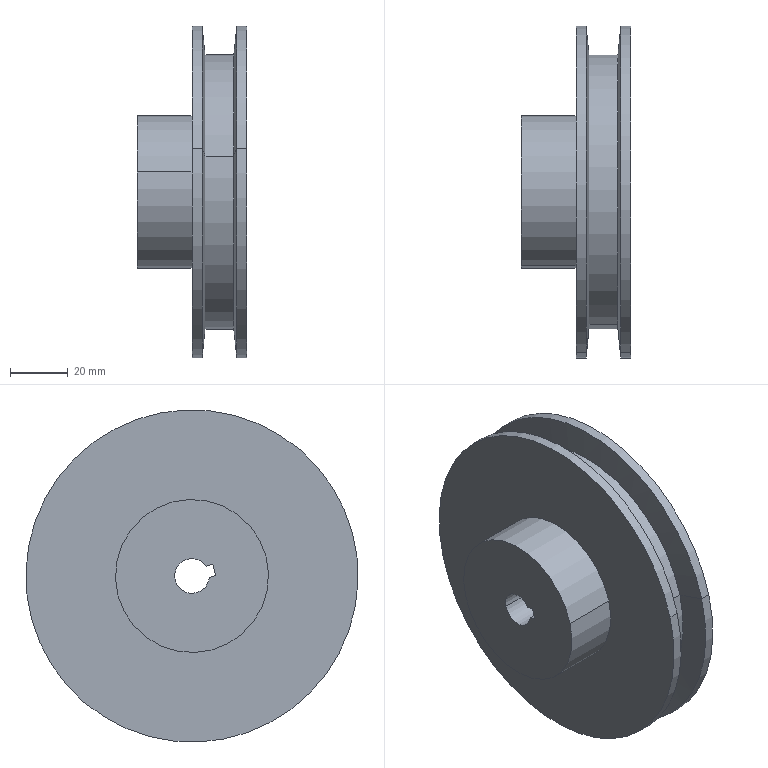Component | SolidWorks | ReducerPulley-1 | 1 solid | 23 faces | box 38 x 115 x 115 mm | volume 149209 mm3 | cylinder 12 | plane 7 | cone 4 | commonest cylinder face diameters 115 x4 12 x2 80 x2 95 x2 53 x2
build123d program:
from build123d import *

# Parameters (mm, degrees)
EXTRUDE1_DEPTH = 87.003


with BuildPart() as part:
    # Sketch1 → Revolve1 (revolve)
    with BuildSketch(Plane.XY, mode=Mode.PRIVATE) as revolve1_sk:
        Polygon((0, 26.5), (19, 26.5), (19, 57.5), (22.5, 57.5), (23.5, 47.5), (33.5, 47.5), (34.5, 57.5), (38, 57.5), (38, 40), (28, 40), (28, 6), (0, 6), align=None)
    revolve(revolve1_sk.sketch.rotate(Axis((28, 0, 0), (1, 0, 0)), 180), axis=Axis((28, 0, 0), (1, 0, 0)))

    # Sketch2 → Extrude1 (cut, through all)
    with BuildSketch(Plane(origin=(28, 0, 0), x_dir=(0, 0, -1), z_dir=(1, 0, 0))):
        Polygon((-2, 8), (2, 8), (2, 2.309), (-2, -3.772), align=None)
    extrude(amount=-EXTRUDE1_DEPTH, mode=Mode.SUBTRACT)


solid = part.part

# Placed as in the assembly
solid = solid.moved(Location((191.216, 175.983, 58.736), (164.849, 0, 0)))
STEP:
#1=COLOUR_RGB('',0.7922,0.8196,0.9333);
#2=FILL_AREA_STYLE_COLOUR('',#1);
#3=FILL_AREA_STYLE('',(#2));
#4=SURFACE_STYLE_FILL_AREA(#3);
#5=SURFACE_SIDE_STYLE('',(#4));
#6=SURFACE_STYLE_USAGE(.BOTH.,#5);
#7=PRESENTATION_STYLE_ASSIGNMENT((#6));
#8=CARTESIAN_POINT('',(8.631,7.156,2.251));
#9=VERTEX_POINT('',#8);
#10=CARTESIAN_POINT('',(8.631,6.693,2.295));
#11=VERTEX_POINT('',#10);
#12=CARTESIAN_POINT('',(8.631,6.928,2.312));
#13=DIRECTION('',(-1.,0.,-0.));
#14=DIRECTION('',(0.,0.9652,-0.2614));
#15=AXIS2_PLACEMENT_3D('',#12,#13,#14);
#16=CIRCLE('',#15,0.2362);
#17=EDGE_CURVE('',#9,#11,#16,.T.);
#18=ORIENTED_EDGE('',*,*,#17,.F.);
#19=CARTESIAN_POINT('',(7.528,7.156,2.251));
#20=VERTEX_POINT('',#19);
#21=CARTESIAN_POINT('',(8.631,7.156,2.251));
#22=DIRECTION('',(-1.,0.,-0.));
#23=VECTOR('',#22,39.37);
#24=LINE('',#21,#23);
#25=EDGE_CURVE('',#9,#20,#24,.T.);
#26=ORIENTED_EDGE('',*,*,#25,.T.);
#27=CARTESIAN_POINT('',(7.528,6.693,2.295));
#28=VERTEX_POINT('',#27);
#29=CARTESIAN_POINT('',(7.528,6.928,2.312));
#30=DIRECTION('',(-1.,0.,-0.));
#31=DIRECTION('',(0.,0.9652,-0.2614));
#32=AXIS2_PLACEMENT_3D('',#29,#30,#31);
#33=CIRCLE('',#32,0.2362);
#34=EDGE_CURVE('',#20,#28,#33,.T.);
#35=ORIENTED_EDGE('',*,*,#34,.T.);
#36=CARTESIAN_POINT('',(8.631,6.693,2.295));
#37=DIRECTION('',(1.,-0.,0.));
#38=VECTOR('',#37,39.37);
#39=LINE('',#36,#38);
#40=EDGE_CURVE('',#28,#11,#39,.T.);
#41=ORIENTED_EDGE('',*,*,#40,.T.);
#42=EDGE_LOOP('',(#18,#26,#35,#41));
#43=FACE_OUTER_BOUND('',#42,.T.);
#44=CARTESIAN_POINT('',(8.631,6.928,2.312));
#45=DIRECTION('',(-1.,0.,-0.));
#46=DIRECTION('',(0.,0.9652,-0.2614));
#47=AXIS2_PLACEMENT_3D('',#44,#45,#46);
#48=CYLINDRICAL_SURFACE('',#47,0.2362);
#49=ADVANCED_FACE('',(#43),#48,.F.);
#50=CARTESIAN_POINT('',(9.024,5.408,2.724));
#51=VERTEX_POINT('',#50);
#52=CARTESIAN_POINT('',(9.024,8.449,1.901));
#53=VERTEX_POINT('',#52);
#54=CARTESIAN_POINT('',(9.024,6.928,2.312));
#55=DIRECTION('',(-1.,0.,-0.));
#56=DIRECTION('',(0.,0.9652,-0.2614));
#57=AXIS2_PLACEMENT_3D('',#54,#55,#56);
#58=CIRCLE('',#57,1.575);
#59=EDGE_CURVE('',#51,#53,#58,.T.);
#60=ORIENTED_EDGE('',*,*,#59,.F.);
#61=CARTESIAN_POINT('',(8.631,5.408,2.724));
#62=VERTEX_POINT('',#61);
#63=CARTESIAN_POINT('',(8.631,5.408,2.724));
#64=DIRECTION('',(-1.,0.,-0.));
#65=VECTOR('',#64,39.37);
#66=LINE('',#63,#65);
#67=EDGE_CURVE('',#51,#62,#66,.T.);
#68=ORIENTED_EDGE('',*,*,#67,.T.);
#69=CARTESIAN_POINT('',(8.631,8.449,1.901));
#70=VERTEX_POINT('',#69);
#71=CARTESIAN_POINT('',(8.631,6.928,2.312));
#72=DIRECTION('',(-1.,0.,-0.));
#73=DIRECTION('',(0.,0.9652,-0.2614));
#74=AXIS2_PLACEMENT_3D('',#71,#72,#73);
#75=CIRCLE('',#74,1.575);
#76=EDGE_CURVE('',#62,#70,#75,.T.);
#77=ORIENTED_EDGE('',*,*,#76,.T.);
#78=CARTESIAN_POINT('',(8.631,8.449,1.901));
#79=DIRECTION('',(-1.,0.,-0.));
#80=VECTOR('',#79,39.37);
#81=LINE('',#78,#80);
#82=EDGE_CURVE('',#53,#70,#81,.T.);
#83=ORIENTED_EDGE('',*,*,#82,.F.);
#84=EDGE_LOOP('',(#60,#68,#77,#83));
#85=FACE_OUTER_BOUND('',#84,.T.);
#86=CARTESIAN_POINT('',(8.631,6.928,2.312));
#87=DIRECTION('',(-1.,0.,-0.));
#88=DIRECTION('',(0.,0.9652,-0.2614));
#89=AXIS2_PLACEMENT_3D('',#86,#87,#88);
#90=CYLINDRICAL_SURFACE('',#89,1.575);
#91=ADVANCED_FACE('',(#85),#90,.F.);
#92=CARTESIAN_POINT('',(9.024,9.114,1.721));
#93=VERTEX_POINT('',#92);
#94=CARTESIAN_POINT('',(9.024,4.743,2.904));
#95=VERTEX_POINT('',#94);
#96=CARTESIAN_POINT('',(9.024,6.928,2.312));
#97=DIRECTION('',(-1.,0.,-0.));
#98=DIRECTION('',(0.,0.9652,-0.2614));
#99=AXIS2_PLACEMENT_3D('',#96,#97,#98);
#100=CIRCLE('',#99,2.264);
#101=EDGE_CURVE('',#93,#95,#100,.T.);
#102=ORIENTED_EDGE('',*,*,#101,.T.);
#103=CARTESIAN_POINT('',(8.886,4.743,2.904));
#104=VERTEX_POINT('',#103);
#105=CARTESIAN_POINT('',(8.631,4.743,2.904));
#106=DIRECTION('',(-1.,0.,-0.));
#107=VECTOR('',#106,39.37);
#108=LINE('',#105,#107);
#109=EDGE_CURVE('',#95,#104,#108,.T.);
#110=ORIENTED_EDGE('',*,*,#109,.T.);
#111=CARTESIAN_POINT('',(8.886,9.114,1.721));
#112=VERTEX_POINT('',#111);
#113=CARTESIAN_POINT('',(8.886,6.928,2.312));
#114=DIRECTION('',(-1.,0.,-0.));
#115=DIRECTION('',(0.,0.9652,-0.2614));
#116=AXIS2_PLACEMENT_3D('',#113,#114,#115);
#117=CIRCLE('',#116,2.264);
#118=EDGE_CURVE('',#112,#104,#117,.T.);
#119=ORIENTED_EDGE('',*,*,#118,.F.);
#120=CARTESIAN_POINT('',(8.631,9.114,1.721));
#121=DIRECTION('',(-1.,0.,-0.));
#122=VECTOR('',#121,39.37);
#123=LINE('',#120,#122);
#124=EDGE_CURVE('',#93,#112,#123,.T.);
#125=ORIENTED_EDGE('',*,*,#124,.F.);
#126=EDGE_LOOP('',(#102,#110,#119,#125));
#127=FACE_OUTER_BOUND('',#126,.T.);
#128=CARTESIAN_POINT('',(8.631,6.928,2.312));
#129=DIRECTION('',(-1.,0.,-0.));
#130=DIRECTION('',(0.,0.9652,-0.2614));
#131=AXIS2_PLACEMENT_3D('',#128,#129,#130);
#132=CYLINDRICAL_SURFACE('',#131,2.264);
#133=ADVANCED_FACE('',(#127),#132,.T.);
#134=CARTESIAN_POINT('',(8.847,8.734,1.824));
#135=VERTEX_POINT('',#134);
#136=CARTESIAN_POINT('',(8.847,5.123,2.801));
#137=VERTEX_POINT('',#136);
#138=CARTESIAN_POINT('',(8.847,6.928,2.312));
#139=DIRECTION('',(-1.,0.,-0.));
#140=DIRECTION('',(0.,0.9652,-0.2614));
#141=AXIS2_PLACEMENT_3D('',#138,#139,#140);
#142=CIRCLE('',#141,1.87);
#143=EDGE_CURVE('',#135,#137,#142,.T.);
#144=ORIENTED_EDGE('',*,*,#143,.F.);
#145=CARTESIAN_POINT('',(8.886,9.114,1.721));
#146=DIRECTION('',(0.0995,0.9604,-0.2601));
#147=VECTOR('',#146,39.37);
#148=LINE('',#145,#147);
#149=EDGE_CURVE('',#135,#112,#148,.T.);
#150=ORIENTED_EDGE('',*,*,#149,.T.);
#151=ORIENTED_EDGE('',*,*,#118,.T.);
#152=CARTESIAN_POINT('',(8.886,4.743,2.904));
#153=DIRECTION('',(0.0995,-0.9604,0.2601));
#154=VECTOR('',#153,39.37);
#155=LINE('',#152,#154);
#156=EDGE_CURVE('',#137,#104,#155,.T.);
#157=ORIENTED_EDGE('',*,*,#156,.F.);
#158=EDGE_LOOP('',(#144,#150,#151,#157));
#159=FACE_OUTER_BOUND('',#158,.T.);
#160=CARTESIAN_POINT('',(8.886,6.928,2.312));
#161=DIRECTION('',(1.,-0.,0.));
#162=DIRECTION('',(0.,-0.9652,0.2614));
#163=AXIS2_PLACEMENT_3D('',#160,#161,#162);
#164=CONICAL_SURFACE('',#163,2.264,1.471);
#165=ADVANCED_FACE('',(#159),#164,.T.);
#166=ORIENTED_EDGE('',*,*,#143,.T.);
#167=CARTESIAN_POINT('',(8.453,5.123,2.801));
#168=VERTEX_POINT('',#167);
#169=CARTESIAN_POINT('',(8.631,5.123,2.801));
#170=DIRECTION('',(-1.,0.,-0.));
#171=VECTOR('',#170,39.37);
#172=LINE('',#169,#171);
#173=EDGE_CURVE('',#137,#168,#172,.T.);
#174=ORIENTED_EDGE('',*,*,#173,.T.);
#175=CARTESIAN_POINT('',(8.453,8.734,1.824));
#176=VERTEX_POINT('',#175);
#177=CARTESIAN_POINT('',(8.453,6.928,2.312));
#178=DIRECTION('',(-1.,0.,-0.));
#179=DIRECTION('',(0.,0.9652,-0.2614));
#180=AXIS2_PLACEMENT_3D('',#177,#178,#179);
#181=CIRCLE('',#180,1.87);
#182=EDGE_CURVE('',#176,#168,#181,.T.);
#183=ORIENTED_EDGE('',*,*,#182,.F.);
#184=CARTESIAN_POINT('',(8.631,8.734,1.824));
#185=DIRECTION('',(-1.,0.,-0.));
#186=VECTOR('',#185,39.37);
#187=LINE('',#184,#186);
#188=EDGE_CURVE('',#135,#176,#187,.T.);
#189=ORIENTED_EDGE('',*,*,#188,.F.);
#190=EDGE_LOOP('',(#166,#174,#183,#189));
#191=FACE_OUTER_BOUND('',#190,.T.);
#192=CARTESIAN_POINT('',(8.631,6.928,2.312));
#193=DIRECTION('',(-1.,0.,-0.));
#194=DIRECTION('',(0.,0.9652,-0.2614));
#195=AXIS2_PLACEMENT_3D('',#192,#193,#194);
#196=CYLINDRICAL_SURFACE('',#195,1.87);
#197=ADVANCED_FACE('',(#191),#196,.T.);
#198=ORIENTED_EDGE('',*,*,#182,.T.);
#199=CARTESIAN_POINT('',(8.414,4.743,2.904));
#200=VERTEX_POINT('',#199);
#201=CARTESIAN_POINT('',(8.453,5.123,2.801));
#202=DIRECTION('',(-0.0995,-0.9604,0.2601));
#203=VECTOR('',#202,39.37);
#204=LINE('',#201,#203);
#205=EDGE_CURVE('',#168,#200,#204,.T.);
#206=ORIENTED_EDGE('',*,*,#205,.T.);
#207=CARTESIAN_POINT('',(8.414,9.114,1.721));
#208=VERTEX_POINT('',#207);
#209=CARTESIAN_POINT('',(8.414,6.928,2.312));
#210=DIRECTION('',(-1.,0.,-0.));
#211=DIRECTION('',(0.,0.9652,-0.2614));
#212=AXIS2_PLACEMENT_3D('',#209,#210,#211);
#213=CIRCLE('',#212,2.264);
#214=EDGE_CURVE('',#208,#200,#213,.T.);
#215=ORIENTED_EDGE('',*,*,#214,.F.);
#216=CARTESIAN_POINT('',(8.453,8.734,1.824));
#217=DIRECTION('',(-0.0995,0.9604,-0.2601));
#218=VECTOR('',#217,39.37);
#219=LINE('',#216,#218);
#220=EDGE_CURVE('',#176,#208,#219,.T.);
#221=ORIENTED_EDGE('',*,*,#220,.F.);
#222=EDGE_LOOP('',(#198,#206,#215,#221));
#223=FACE_OUTER_BOUND('',#222,.T.);
#224=CARTESIAN_POINT('',(8.453,6.928,2.312));
#225=DIRECTION('',(-1.,0.,-0.));
#226=DIRECTION('',(0.,0.9652,-0.2614));
#227=AXIS2_PLACEMENT_3D('',#224,#225,#226);
#228=CONICAL_SURFACE('',#227,1.87,1.471);
#229=ADVANCED_FACE('',(#223),#228,.T.);
#230=ORIENTED_EDGE('',*,*,#214,.T.);
#231=CARTESIAN_POINT('',(8.276,4.743,2.904));
#232=VERTEX_POINT('',#231);
#233=CARTESIAN_POINT('',(8.631,4.743,2.904));
#234=DIRECTION('',(-1.,0.,-0.));
#235=VECTOR('',#234,39.37);
#236=LINE('',#233,#235);
#237=EDGE_CURVE('',#200,#232,#236,.T.);
#238=ORIENTED_EDGE('',*,*,#237,.T.);
#239=CARTESIAN_POINT('',(8.276,9.114,1.721));
#240=VERTEX_POINT('',#239);
#241=CARTESIAN_POINT('',(8.276,6.928,2.312));
#242=DIRECTION('',(-1.,0.,-0.));
#243=DIRECTION('',(0.,0.9652,-0.2614));
#244=AXIS2_PLACEMENT_3D('',#241,#242,#243);
#245=CIRCLE('',#244,2.264);
#246=EDGE_CURVE('',#240,#232,#245,.T.);
#247=ORIENTED_EDGE('',*,*,#246,.F.);
#248=CARTESIAN_POINT('',(8.631,9.114,1.721));
#249=DIRECTION('',(-1.,0.,-0.));
#250=VECTOR('',#249,39.37);
#251=LINE('',#248,#250);
#252=EDGE_CURVE('',#208,#240,#251,.T.);
#253=ORIENTED_EDGE('',*,*,#252,.F.);
#254=EDGE_LOOP('',(#230,#238,#247,#253));
#255=FACE_OUTER_BOUND('',#254,.T.);
#256=CARTESIAN_POINT('',(8.631,6.928,2.312));
#257=DIRECTION('',(-1.,0.,-0.));
#258=DIRECTION('',(0.,0.9652,-0.2614));
#259=AXIS2_PLACEMENT_3D('',#256,#257,#258);
#260=CYLINDRICAL_SURFACE('',#259,2.264);
#261=ADVANCED_FACE('',(#255),#260,.T.);
#262=CARTESIAN_POINT('',(8.276,7.936,2.04));
#263=VERTEX_POINT('',#262);
#264=CARTESIAN_POINT('',(8.276,5.921,2.585));
#265=VERTEX_POINT('',#264);
#266=CARTESIAN_POINT('',(8.276,6.928,2.312));
#267=DIRECTION('',(-1.,0.,-0.));
#268=DIRECTION('',(0.,0.9652,-0.2614));
#269=AXIS2_PLACEMENT_3D('',#266,#267,#268);
#270=CIRCLE('',#269,1.043);
#271=EDGE_CURVE('',#263,#265,#270,.T.);
#272=ORIENTED_EDGE('',*,*,#271,.T.);
#273=CARTESIAN_POINT('',(7.528,5.921,2.585));
#274=VERTEX_POINT('',#273);
#275=CARTESIAN_POINT('',(8.631,5.921,2.585));
#276=DIRECTION('',(-1.,0.,-0.));
#277=VECTOR('',#276,39.37);
#278=LINE('',#275,#277);
#279=EDGE_CURVE('',#265,#274,#278,.T.);
#280=ORIENTED_EDGE('',*,*,#279,.T.);
#281=CARTESIAN_POINT('',(7.528,7.936,2.04));
#282=VERTEX_POINT('',#281);
#283=CARTESIAN_POINT('',(7.528,6.928,2.312));
#284=DIRECTION('',(-1.,0.,-0.));
#285=DIRECTION('',(0.,0.9652,-0.2614));
#286=AXIS2_PLACEMENT_3D('',#283,#284,#285);
#287=CIRCLE('',#286,1.043);
#288=EDGE_CURVE('',#282,#274,#287,.T.);
#289=ORIENTED_EDGE('',*,*,#288,.F.);
#290=CARTESIAN_POINT('',(8.631,7.936,2.04));
#291=DIRECTION('',(-1.,0.,-0.));
#292=VECTOR('',#291,39.37);
#293=LINE('',#290,#292);
#294=EDGE_CURVE('',#263,#282,#293,.T.);
#295=ORIENTED_EDGE('',*,*,#294,.F.);
#296=EDGE_LOOP('',(#272,#280,#289,#295));
#297=FACE_OUTER_BOUND('',#296,.T.);
#298=CARTESIAN_POINT('',(8.631,6.928,2.312));
#299=DIRECTION('',(-1.,0.,-0.));
#300=DIRECTION('',(0.,0.9652,-0.2614));
#301=AXIS2_PLACEMENT_3D('',#298,#299,#300);
#302=CYLINDRICAL_SURFACE('',#301,1.043);
#303=ADVANCED_FACE('',(#297),#302,.T.);
#304=CARTESIAN_POINT('',(7.528,6.645,2.471));
#305=VERTEX_POINT('',#304);
#306=CARTESIAN_POINT('',(7.528,6.604,2.319));
#307=VERTEX_POINT('',#306);
#308=CARTESIAN_POINT('',(7.528,6.604,2.319));
#309=DIRECTION('',(-0.,-0.2614,-0.9652));
#310=VECTOR('',#309,39.37);
#311=LINE('',#308,#310);
#312=EDGE_CURVE('',#305,#307,#311,.T.);
#313=ORIENTED_EDGE('',*,*,#312,.T.);
#314=CARTESIAN_POINT('',(7.528,6.604,2.319));
#315=DIRECTION('',(0.,0.9652,-0.2614));
#316=VECTOR('',#315,39.37);
#317=LINE('',#314,#316);
#318=EDGE_CURVE('',#307,#28,#317,.T.);
#319=ORIENTED_EDGE('',*,*,#318,.T.);
#320=ORIENTED_EDGE('',*,*,#34,.F.);
#321=CARTESIAN_POINT('',(7.528,6.734,2.447));
#322=VERTEX_POINT('',#321);
#323=CARTESIAN_POINT('',(7.528,6.928,2.312));
#324=DIRECTION('',(-1.,0.,-0.));
#325=DIRECTION('',(0.,0.9652,-0.2614));
#326=AXIS2_PLACEMENT_3D('',#323,#324,#325);
#327=CIRCLE('',#326,0.2362);
#328=EDGE_CURVE('',#322,#20,#327,.T.);
#329=ORIENTED_EDGE('',*,*,#328,.F.);
#330=CARTESIAN_POINT('',(7.528,6.645,2.471));
#331=DIRECTION('',(-0.,-0.9652,0.2614));
#332=VECTOR('',#331,39.37);
#333=LINE('',#330,#332);
#334=EDGE_CURVE('',#322,#305,#333,.T.);
#335=ORIENTED_EDGE('',*,*,#334,.T.);
#336=EDGE_LOOP('',(#313,#319,#320,#329,#335));
#337=FACE_BOUND('',#336,.T.);
#338=ORIENTED_EDGE('',*,*,#288,.T.);
#339=CARTESIAN_POINT('',(7.528,6.928,2.312));
#340=DIRECTION('',(-1.,0.,-0.));
#341=DIRECTION('',(0.,0.9652,-0.2614));
#342=AXIS2_PLACEMENT_3D('',#339,#340,#341);
#343=CIRCLE('',#342,1.043);
#344=EDGE_CURVE('',#274,#282,#343,.T.);
#345=ORIENTED_EDGE('',*,*,#344,.T.);
#346=EDGE_LOOP('',(#338,#345));
#347=FACE_OUTER_BOUND('',#346,.T.);
#348=CARTESIAN_POINT('',(7.528,6.7,2.374));
#349=DIRECTION('',(1.,-0.,0.));
#350=DIRECTION('',(-0.,-0.9652,0.2614));
#351=AXIS2_PLACEMENT_3D('',#348,#349,#350);
#352=PLANE('',#351);
#353=ADVANCED_FACE('',(#337,#347),#352,.F.);
#354=ORIENTED_EDGE('',*,*,#279,.F.);
#355=CARTESIAN_POINT('',(8.276,6.928,2.312));
#356=DIRECTION('',(-1.,0.,-0.));
#357=DIRECTION('',(0.,0.9652,-0.2614));
#358=AXIS2_PLACEMENT_3D('',#355,#356,#357);
#359=CIRCLE('',#358,1.043);
#360=EDGE_CURVE('',#265,#263,#359,.T.);
#361=ORIENTED_EDGE('',*,*,#360,.T.);
#362=ORIENTED_EDGE('',*,*,#294,.T.);
#363=ORIENTED_EDGE('',*,*,#344,.F.);
#364=EDGE_LOOP('',(#354,#361,#362,#363));
#365=FACE_OUTER_BOUND('',#364,.T.);
#366=CARTESIAN_POINT('',(8.631,6.928,2.312));
#367=DIRECTION('',(-1.,0.,-0.));
#368=DIRECTION('',(0.,0.9652,-0.2614));
#369=AXIS2_PLACEMENT_3D('',#366,#367,#368);
#370=CYLINDRICAL_SURFACE('',#369,1.043);
#371=ADVANCED_FACE('',(#365),#370,.T.);
#372=ORIENTED_EDGE('',*,*,#271,.F.);
#373=ORIENTED_EDGE('',*,*,#360,.F.);
#374=EDGE_LOOP('',(#372,#373));
#375=FACE_BOUND('',#374,.T.);
#376=ORIENTED_EDGE('',*,*,#246,.T.);
#377=CARTESIAN_POINT('',(8.276,6.928,2.312));
#378=DIRECTION('',(-1.,0.,-0.));
#379=DIRECTION('',(0.,0.9652,-0.2614));
#380=AXIS2_PLACEMENT_3D('',#377,#378,#379);
#381=CIRCLE('',#380,2.264);
#382=EDGE_CURVE('',#232,#240,#381,.T.);
#383=ORIENTED_EDGE('',*,*,#382,.T.);
#384=EDGE_LOOP('',(#376,#383));
#385=FACE_OUTER_BOUND('',#384,.T.);
#386=CARTESIAN_POINT('',(8.276,5.921,2.585));
#387=DIRECTION('',(1.,-0.,0.));
#388=DIRECTION('',(-0.,-0.9652,0.2614));
#389=AXIS2_PLACEMENT_3D('',#386,#387,#388);
#390=PLANE('',#389);
#391=ADVANCED_FACE('',(#375,#385),#390,.F.);
#392=ORIENTED_EDGE('',*,*,#237,.F.);
#393=CARTESIAN_POINT('',(8.414,6.928,2.312));
#394=DIRECTION('',(-1.,0.,-0.));
#395=DIRECTION('',(0.,0.9652,-0.2614));
#396=AXIS2_PLACEMENT_3D('',#393,#394,#395);
#397=CIRCLE('',#396,2.264);
#398=EDGE_CURVE('',#200,#208,#397,.T.);
#399=ORIENTED_EDGE('',*,*,#398,.T.);
#400=ORIENTED_EDGE('',*,*,#252,.T.);
#401=ORIENTED_EDGE('',*,*,#382,.F.);
#402=EDGE_LOOP('',(#392,#399,#400,#401));
#403=FACE_OUTER_BOUND('',#402,.T.);
#404=CARTESIAN_POINT('',(8.631,6.928,2.312));
#405=DIRECTION('',(-1.,0.,-0.));
#406=DIRECTION('',(0.,0.9652,-0.2614));
#407=AXIS2_PLACEMENT_3D('',#404,#405,#406);
#408=CYLINDRICAL_SURFACE('',#407,2.264);
#409=ADVANCED_FACE('',(#403),#408,.T.);
#410=ORIENTED_EDGE('',*,*,#205,.F.);
#411=CARTESIAN_POINT('',(8.453,6.928,2.312));
#412=DIRECTION('',(-1.,0.,-0.));
#413=DIRECTION('',(0.,0.9652,-0.2614));
#414=AXIS2_PLACEMENT_3D('',#411,#412,#413);
#415=CIRCLE('',#414,1.87);
#416=EDGE_CURVE('',#168,#176,#415,.T.);
#417=ORIENTED_EDGE('',*,*,#416,.T.);
#418=ORIENTED_EDGE('',*,*,#220,.T.);
#419=ORIENTED_EDGE('',*,*,#398,.F.);
#420=EDGE_LOOP('',(#410,#417,#418,#419));
#421=FACE_OUTER_BOUND('',#420,.T.);
#422=CARTESIAN_POINT('',(8.453,6.928,2.312));
#423=DIRECTION('',(-1.,0.,-0.));
#424=DIRECTION('',(0.,0.9652,-0.2614));
#425=AXIS2_PLACEMENT_3D('',#422,#423,#424);
#426=CONICAL_SURFACE('',#425,1.87,1.471);
#427=ADVANCED_FACE('',(#421),#426,.T.);
#428=ORIENTED_EDGE('',*,*,#173,.F.);
#429=CARTESIAN_POINT('',(8.847,6.928,2.312));
#430=DIRECTION('',(-1.,0.,-0.));
#431=DIRECTION('',(0.,0.9652,-0.2614));
#432=AXIS2_PLACEMENT_3D('',#429,#430,#431);
#433=CIRCLE('',#432,1.87);
#434=EDGE_CURVE('',#137,#135,#433,.T.);
#435=ORIENTED_EDGE('',*,*,#434,.T.);
#436=ORIENTED_EDGE('',*,*,#188,.T.);
#437=ORIENTED_EDGE('',*,*,#416,.F.);
#438=EDGE_LOOP('',(#428,#435,#436,#437));
#439=FACE_OUTER_BOUND('',#438,.T.);
#440=CARTESIAN_POINT('',(8.631,6.928,2.312));
#441=DIRECTION('',(-1.,0.,-0.));
#442=DIRECTION('',(0.,0.9652,-0.2614));
#443=AXIS2_PLACEMENT_3D('',#440,#441,#442);
#444=CYLINDRICAL_SURFACE('',#443,1.87);
#445=ADVANCED_FACE('',(#439),#444,.T.);
#446=ORIENTED_EDGE('',*,*,#149,.F.);
#447=ORIENTED_EDGE('',*,*,#434,.F.);
#448=ORIENTED_EDGE('',*,*,#156,.T.);
#449=CARTESIAN_POINT('',(8.886,6.928,2.312));
#450=DIRECTION('',(-1.,0.,-0.));
#451=DIRECTION('',(0.,0.9652,-0.2614));
#452=AXIS2_PLACEMENT_3D('',#449,#450,#451);
#453=CIRCLE('',#452,2.264);
#454=EDGE_CURVE('',#104,#112,#453,.T.);
#455=ORIENTED_EDGE('',*,*,#454,.T.);
#456=EDGE_LOOP('',(#446,#447,#448,#455));
#457=FACE_OUTER_BOUND('',#456,.T.);
#458=CARTESIAN_POINT('',(8.886,6.928,2.312));
#459=DIRECTION('',(1.,-0.,0.));
#460=DIRECTION('',(0.,-0.9652,0.2614));
#461=AXIS2_PLACEMENT_3D('',#458,#459,#460);
#462=CONICAL_SURFACE('',#461,2.264,1.471);
#463=ADVANCED_FACE('',(#457),#462,.T.);
#464=ORIENTED_EDGE('',*,*,#109,.F.);
#465=CARTESIAN_POINT('',(9.024,6.928,2.312));
#466=DIRECTION('',(-1.,0.,-0.));
#467=DIRECTION('',(0.,0.9652,-0.2614));
#468=AXIS2_PLACEMENT_3D('',#465,#466,#467);
#469=CIRCLE('',#468,2.264);
#470=EDGE_CURVE('',#95,#93,#469,.T.);
#471=ORIENTED_EDGE('',*,*,#470,.T.);
#472=ORIENTED_EDGE('',*,*,#124,.T.);
#473=ORIENTED_EDGE('',*,*,#454,.F.);
#474=EDGE_LOOP('',(#464,#471,#472,#473));
#475=FACE_OUTER_BOUND('',#474,.T.);
#476=CARTESIAN_POINT('',(8.631,6.928,2.312));
#477=DIRECTION('',(-1.,0.,-0.));
#478=DIRECTION('',(0.,0.9652,-0.2614));
#479=AXIS2_PLACEMENT_3D('',#476,#477,#478);
#480=CYLINDRICAL_SURFACE('',#479,2.264);
#481=ADVANCED_FACE('',(#475),#480,.T.);
#482=ORIENTED_EDGE('',*,*,#101,.F.);
#483=ORIENTED_EDGE('',*,*,#470,.F.);
#484=EDGE_LOOP('',(#482,#483));
#485=FACE_OUTER_BOUND('',#484,.T.);
#486=CARTESIAN_POINT('',(9.024,6.928,2.312));
#487=DIRECTION('',(-1.,0.,-0.));
#488=DIRECTION('',(0.,0.9652,-0.2614));
#489=AXIS2_PLACEMENT_3D('',#486,#487,#488);
#490=CIRCLE('',#489,1.575);
#491=EDGE_CURVE('',#53,#51,#490,.T.);
#492=ORIENTED_EDGE('',*,*,#491,.T.);
#493=ORIENTED_EDGE('',*,*,#59,.T.);
#494=EDGE_LOOP('',(#492,#493));
#495=FACE_BOUND('',#494,.T.);
#496=CARTESIAN_POINT('',(9.024,4.743,2.904));
#497=DIRECTION('',(-1.,0.,-0.));
#498=DIRECTION('',(0.,0.9652,-0.2614));
#499=AXIS2_PLACEMENT_3D('',#496,#497,#498);
#500=PLANE('',#499);
#501=ADVANCED_FACE('',(#485,#495),#500,.F.);
#502=ORIENTED_EDGE('',*,*,#67,.F.);
#503=ORIENTED_EDGE('',*,*,#491,.F.);
#504=ORIENTED_EDGE('',*,*,#82,.T.);
#505=CARTESIAN_POINT('',(8.631,6.928,2.312));
#506=DIRECTION('',(-1.,0.,-0.));
#507=DIRECTION('',(0.,0.9652,-0.2614));
#508=AXIS2_PLACEMENT_3D('',#505,#506,#507);
#509=CIRCLE('',#508,1.575);
#510=EDGE_CURVE('',#70,#62,#509,.T.);
#511=ORIENTED_EDGE('',*,*,#510,.T.);
#512=EDGE_LOOP('',(#502,#503,#504,#511));
#513=FACE_OUTER_BOUND('',#512,.T.);
#514=CARTESIAN_POINT('',(8.631,6.928,2.312));
#515=DIRECTION('',(-1.,0.,-0.));
#516=DIRECTION('',(0.,0.9652,-0.2614));
#517=AXIS2_PLACEMENT_3D('',#514,#515,#516);
#518=CYLINDRICAL_SURFACE('',#517,1.575);
#519=ADVANCED_FACE('',(#513),#518,.F.);
#520=ORIENTED_EDGE('',*,*,#510,.F.);
#521=ORIENTED_EDGE('',*,*,#76,.F.);
#522=EDGE_LOOP('',(#520,#521));
#523=FACE_OUTER_BOUND('',#522,.T.);
#524=CARTESIAN_POINT('',(8.631,6.734,2.447));
#525=VERTEX_POINT('',#524);
#526=CARTESIAN_POINT('',(8.631,6.928,2.312));
#527=DIRECTION('',(-1.,0.,-0.));
#528=DIRECTION('',(0.,0.9652,-0.2614));
#529=AXIS2_PLACEMENT_3D('',#526,#527,#528);
#530=CIRCLE('',#529,0.2362);
#531=EDGE_CURVE('',#525,#9,#530,.T.);
#532=ORIENTED_EDGE('',*,*,#531,.T.);
#533=ORIENTED_EDGE('',*,*,#17,.T.);
#534=CARTESIAN_POINT('',(8.631,6.604,2.319));
#535=VERTEX_POINT('',#534);
#536=CARTESIAN_POINT('',(8.631,6.604,2.319));
#537=DIRECTION('',(0.,0.9652,-0.2614));
#538=VECTOR('',#537,39.37);
#539=LINE('',#536,#538);
#540=EDGE_CURVE('',#535,#11,#539,.T.);
#541=ORIENTED_EDGE('',*,*,#540,.F.);
#542=CARTESIAN_POINT('',(8.631,6.645,2.471));
#543=VERTEX_POINT('',#542);
#544=CARTESIAN_POINT('',(8.631,6.604,2.319));
#545=DIRECTION('',(-0.,-0.2614,-0.9652));
#546=VECTOR('',#545,39.37);
#547=LINE('',#544,#546);
#548=EDGE_CURVE('',#543,#535,#547,.T.);
#549=ORIENTED_EDGE('',*,*,#548,.F.);
#550=CARTESIAN_POINT('',(8.631,6.645,2.471));
#551=DIRECTION('',(-0.,-0.9652,0.2614));
#552=VECTOR('',#551,39.37);
#553=LINE('',#550,#552);
#554=EDGE_CURVE('',#525,#543,#553,.T.);
#555=ORIENTED_EDGE('',*,*,#554,.F.);
#556=EDGE_LOOP('',(#532,#533,#541,#549,#555));
#557=FACE_BOUND('',#556,.T.);
#558=CARTESIAN_POINT('',(8.631,5.408,2.724));
#559=DIRECTION('',(-1.,0.,-0.));
#560=DIRECTION('',(0.,0.9652,-0.2614));
#561=AXIS2_PLACEMENT_3D('',#558,#559,#560);
#562=PLANE('',#561);
#563=ADVANCED_FACE('',(#523,#557),#562,.F.);
#564=ORIENTED_EDGE('',*,*,#25,.F.);
#565=ORIENTED_EDGE('',*,*,#531,.F.);
#566=CARTESIAN_POINT('',(8.631,6.734,2.447));
#567=DIRECTION('',(-1.,0.,-0.));
#568=VECTOR('',#567,39.37);
#569=LINE('',#566,#568);
#570=EDGE_CURVE('',#525,#322,#569,.T.);
#571=ORIENTED_EDGE('',*,*,#570,.T.);
#572=ORIENTED_EDGE('',*,*,#328,.T.);
#573=EDGE_LOOP('',(#564,#565,#571,#572));
#574=FACE_OUTER_BOUND('',#573,.T.);
#575=CARTESIAN_POINT('',(8.631,6.928,2.312));
#576=DIRECTION('',(-1.,0.,-0.));
#577=DIRECTION('',(0.,0.9652,-0.2614));
#578=AXIS2_PLACEMENT_3D('',#575,#576,#577);
#579=CYLINDRICAL_SURFACE('',#578,0.2362);
#580=ADVANCED_FACE('',(#574),#579,.F.);
#581=ORIENTED_EDGE('',*,*,#318,.F.);
#582=CARTESIAN_POINT('',(7.528,6.604,2.319));
#583=DIRECTION('',(1.,-0.,0.));
#584=VECTOR('',#583,39.37);
#585=LINE('',#582,#584);
#586=EDGE_CURVE('',#307,#535,#585,.T.);
#587=ORIENTED_EDGE('',*,*,#586,.T.);
#588=ORIENTED_EDGE('',*,*,#540,.T.);
#589=ORIENTED_EDGE('',*,*,#40,.F.);
#590=EDGE_LOOP('',(#581,#587,#588,#589));
#591=FACE_OUTER_BOUND('',#590,.T.);
#592=CARTESIAN_POINT('',(7.528,6.604,2.319));
#593=DIRECTION('',(-0.,-0.2614,-0.9652));
#594=DIRECTION('',(0.,0.9652,-0.2614));
#595=AXIS2_PLACEMENT_3D('',#592,#593,#594);
#596=PLANE('',#595);
#597=ADVANCED_FACE('',(#591),#596,.F.);
#598=ORIENTED_EDGE('',*,*,#554,.T.);
#599=CARTESIAN_POINT('',(7.528,6.645,2.471));
#600=DIRECTION('',(1.,-0.,0.));
#601=VECTOR('',#600,39.37);
#602=LINE('',#599,#601);
#603=EDGE_CURVE('',#305,#543,#602,.T.);
#604=ORIENTED_EDGE('',*,*,#603,.F.);
#605=ORIENTED_EDGE('',*,*,#334,.F.);
#606=ORIENTED_EDGE('',*,*,#570,.F.);
#607=EDGE_LOOP('',(#598,#604,#605,#606));
#608=FACE_OUTER_BOUND('',#607,.T.);
#609=CARTESIAN_POINT('',(7.528,6.645,2.471));
#610=DIRECTION('',(0.,0.2614,0.9652));
#611=DIRECTION('',(-0.,-0.9652,0.2614));
#612=AXIS2_PLACEMENT_3D('',#609,#610,#611);
#613=PLANE('',#612);
#614=ADVANCED_FACE('',(#608),#613,.F.);
#615=ORIENTED_EDGE('',*,*,#548,.T.);
#616=ORIENTED_EDGE('',*,*,#586,.F.);
#617=ORIENTED_EDGE('',*,*,#312,.F.);
#618=ORIENTED_EDGE('',*,*,#603,.T.);
#619=EDGE_LOOP('',(#615,#616,#617,#618));
#620=FACE_OUTER_BOUND('',#619,.T.);
#621=CARTESIAN_POINT('',(7.528,6.604,2.319));
#622=DIRECTION('',(-0.,-0.9652,0.2614));
#623=DIRECTION('',(-1.,0.,-0.));
#624=AXIS2_PLACEMENT_3D('',#621,#622,#623);
#625=PLANE('',#624);
#626=ADVANCED_FACE('',(#620),#625,.F.);
#627=CLOSED_SHELL('',(#49,#91,#133,#165,#197,#229,#261,#303,#353,#371,#391,#409,#427,#445,#463,#481,#501,#519,#563,#580,#597,#614,#626));
#628=MANIFOLD_SOLID_BREP('',#627);
#629=STYLED_ITEM('',(#7),#628);
#630=(LENGTH_UNIT()NAMED_UNIT(*)SI_UNIT($,.METRE.));
#631=LENGTH_MEASURE_WITH_UNIT(LENGTH_MEASURE(0.0254),#630);
#632=DIMENSIONAL_EXPONENTS(1.,0.,0.,0.,0.,0.,0.);
#633=(CONVERSION_BASED_UNIT('',#631)LENGTH_UNIT()NAMED_UNIT(#632));
#634=UNCERTAINTY_MEASURE_WITH_UNIT(LENGTH_MEASURE(0.00001),#633,'','');
#635=(NAMED_UNIT(*)PLANE_ANGLE_UNIT()SI_UNIT($,.RADIAN.));
#636=(NAMED_UNIT(*)SI_UNIT($,.STERADIAN.)SOLID_ANGLE_UNIT());
#637=(GEOMETRIC_REPRESENTATION_CONTEXT(3)GLOBAL_UNCERTAINTY_ASSIGNED_CONTEXT((#634))GLOBAL_UNIT_ASSIGNED_CONTEXT((#633,#635,#636))REPRESENTATION_CONTEXT('',''));
#638=MECHANICAL_DESIGN_GEOMETRIC_PRESENTATION_REPRESENTATION('',(#629),#637);
#639=CARTESIAN_POINT('',(0.,0.,0.));
#640=DIRECTION('',(0.,0.,1.));
#641=DIRECTION('',(1.,0.,0.));
#642=AXIS2_PLACEMENT_3D('',#639,#640,#641);
#643=(LENGTH_UNIT()NAMED_UNIT(*)SI_UNIT($,.METRE.));
#644=LENGTH_MEASURE_WITH_UNIT(LENGTH_MEASURE(0.0254),#643);
#645=DIMENSIONAL_EXPONENTS(1.,0.,0.,0.,0.,0.,0.);
#646=(CONVERSION_BASED_UNIT('',#644)LENGTH_UNIT()NAMED_UNIT(#645));
#647=UNCERTAINTY_MEASURE_WITH_UNIT(LENGTH_MEASURE(0.00001),#646,'','');
#648=(NAMED_UNIT(*)PLANE_ANGLE_UNIT()SI_UNIT($,.RADIAN.));
#649=(NAMED_UNIT(*)SI_UNIT($,.STERADIAN.)SOLID_ANGLE_UNIT());
#650=(GEOMETRIC_REPRESENTATION_CONTEXT(3)GLOBAL_UNCERTAINTY_ASSIGNED_CONTEXT((#647))GLOBAL_UNIT_ASSIGNED_CONTEXT((#646,#648,#649))REPRESENTATION_CONTEXT('',''));
#651=ADVANCED_BREP_SHAPE_REPRESENTATION('',(#628,#642),#650);
#652=PRESENTATION_LAYER_ASSIGNMENT('','',(#629));